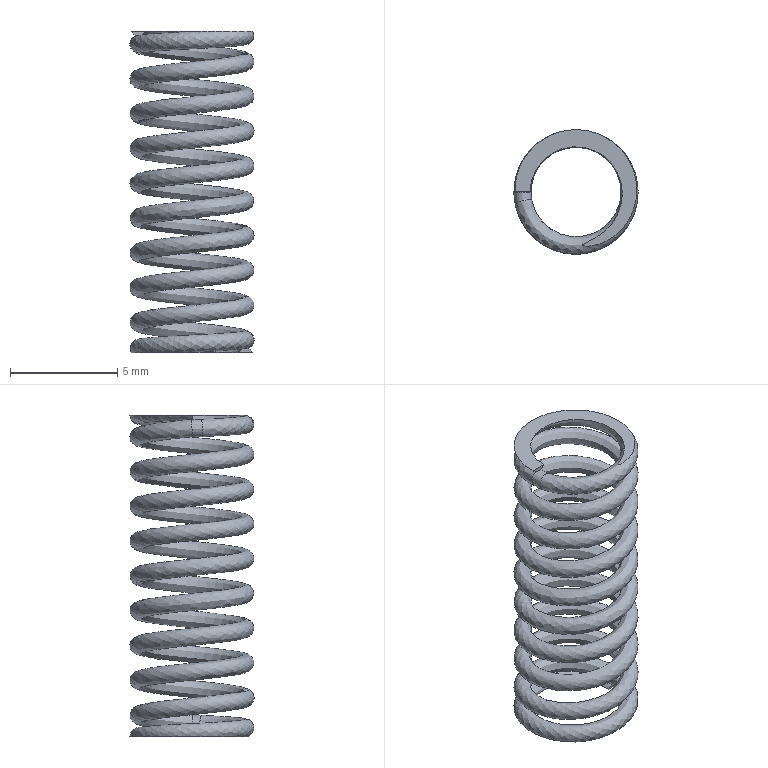Component | NX | DXF_03_COMPRESSION_SPRING | 1 solid | 9 faces | volume 79 mm3 | spline 5 | plane 4